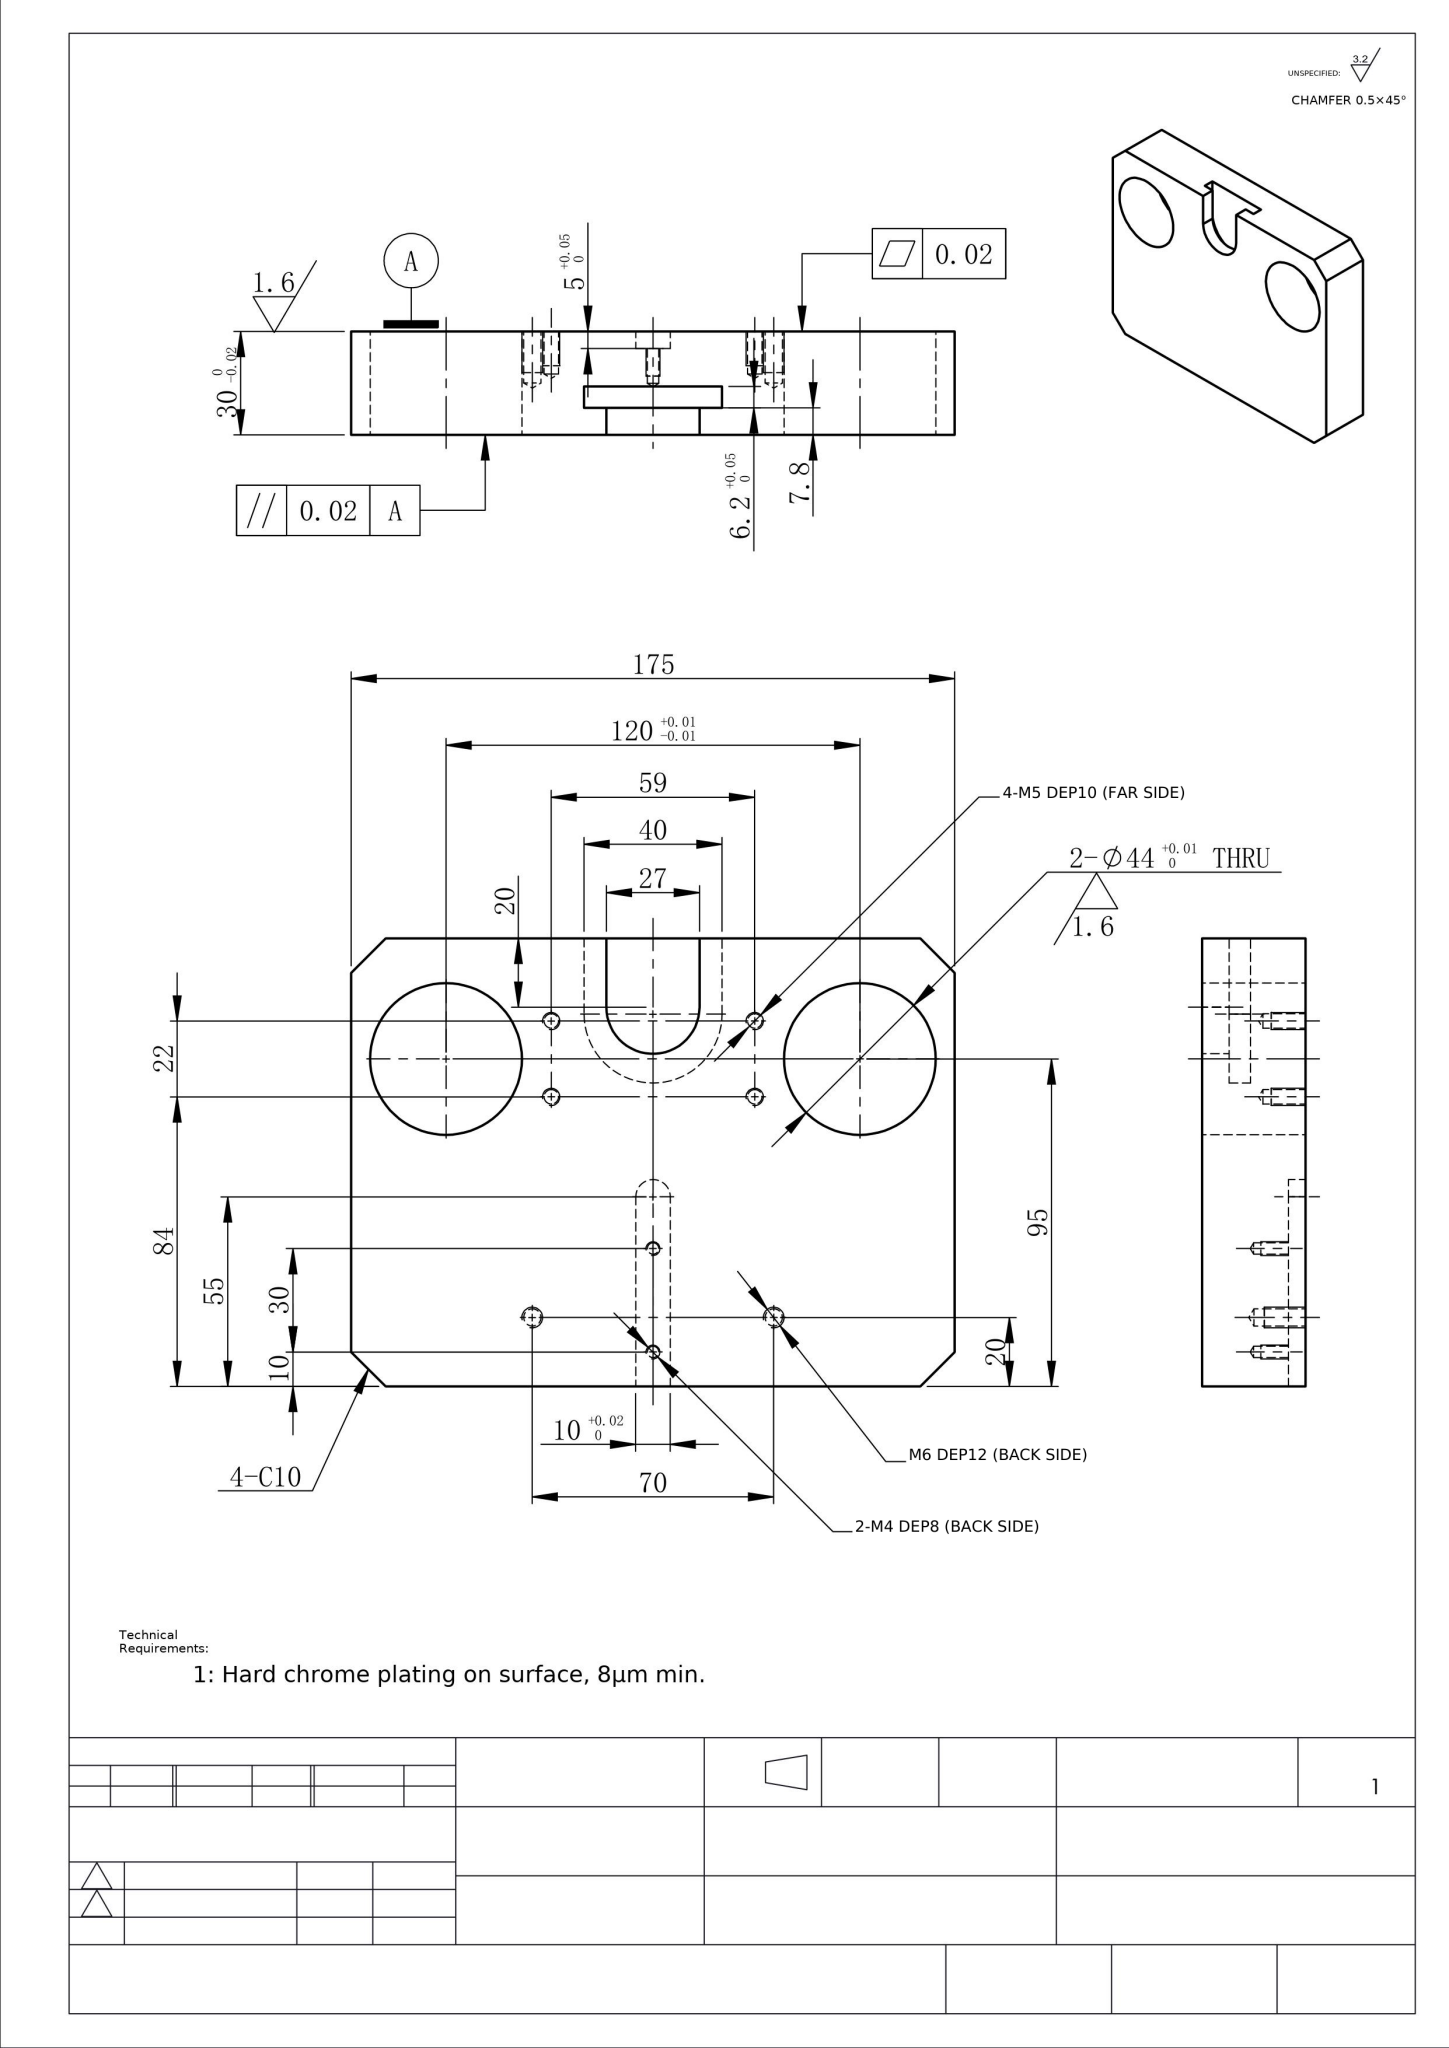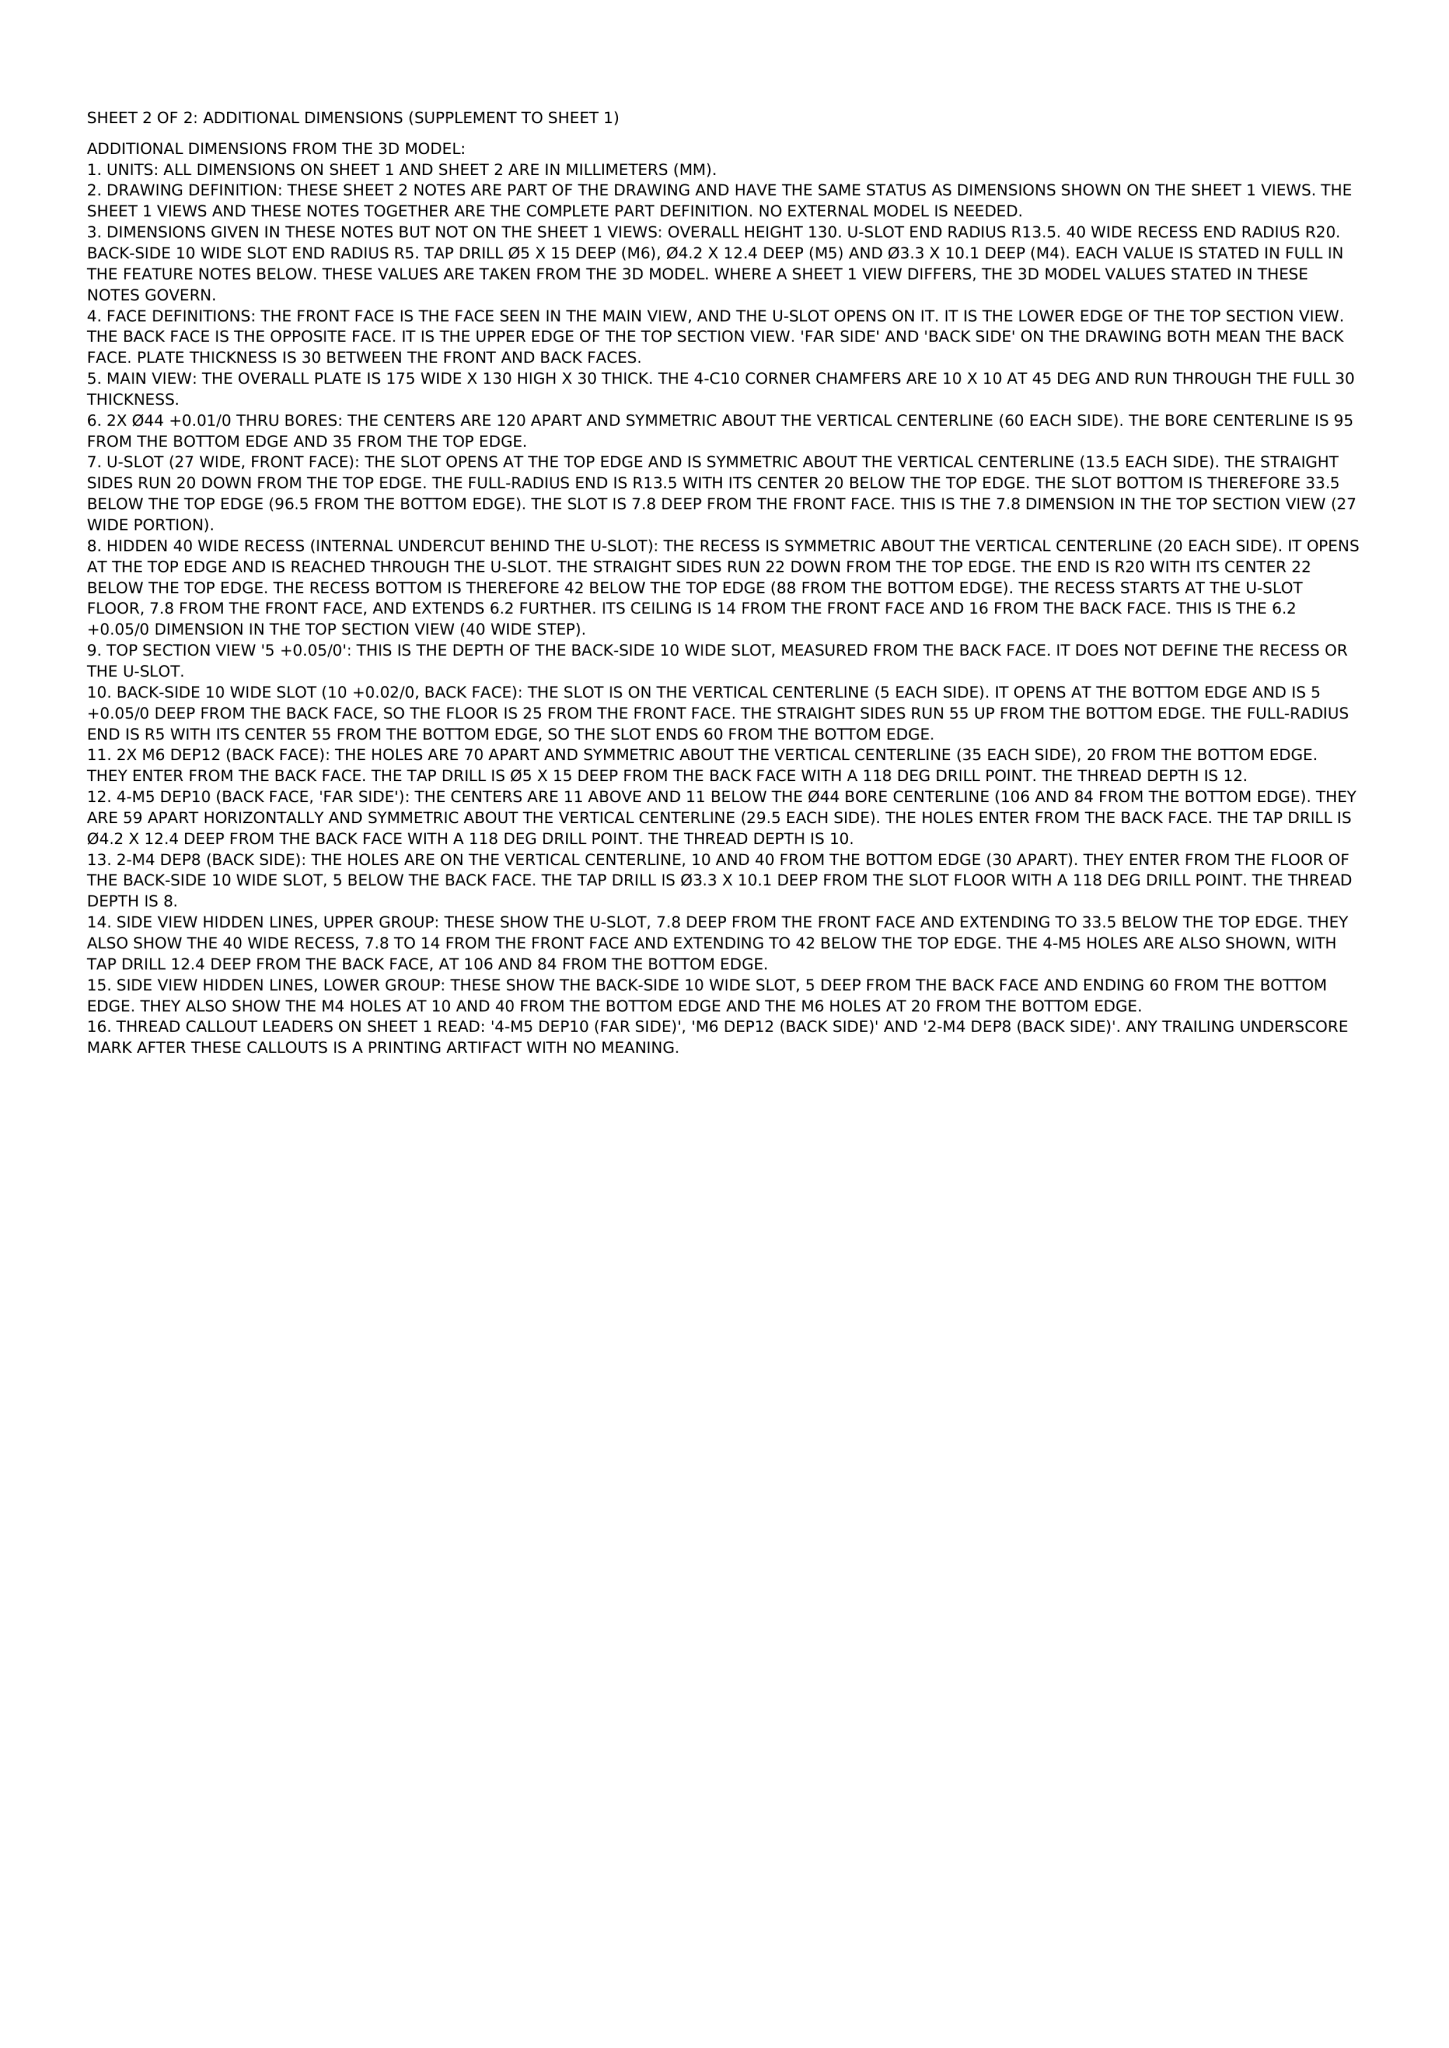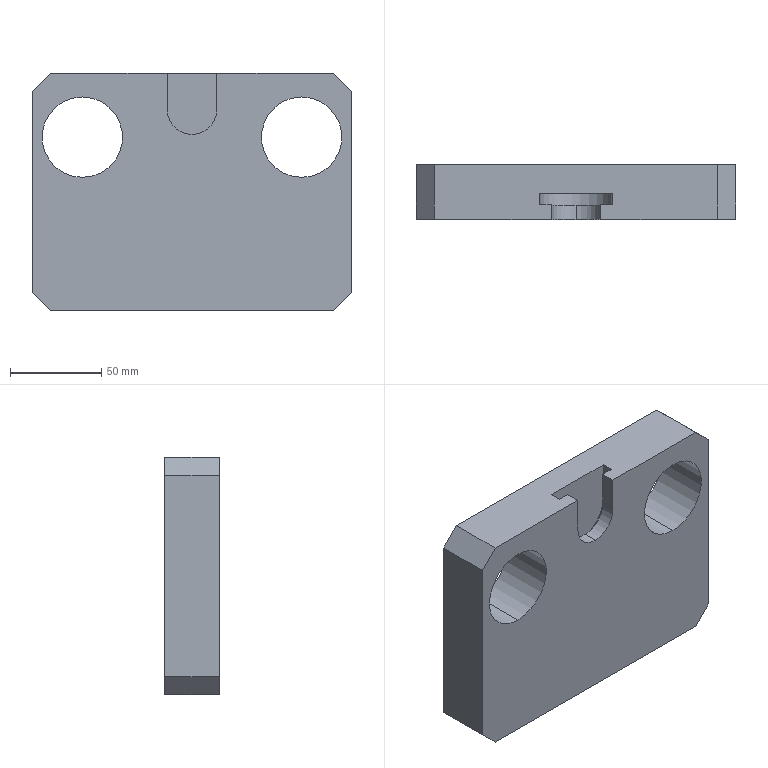Part | NX | mm | 1 solid | 60 faces | box 175 x 30 x 130 mm | volume 565028 mm3 | cylinder 25 | plane 19 | cone 16 | commonest cylinder face diameters 4.2 x8 5 x4 3.3 x4 44 x4 27 x2 10 x2 40 x1